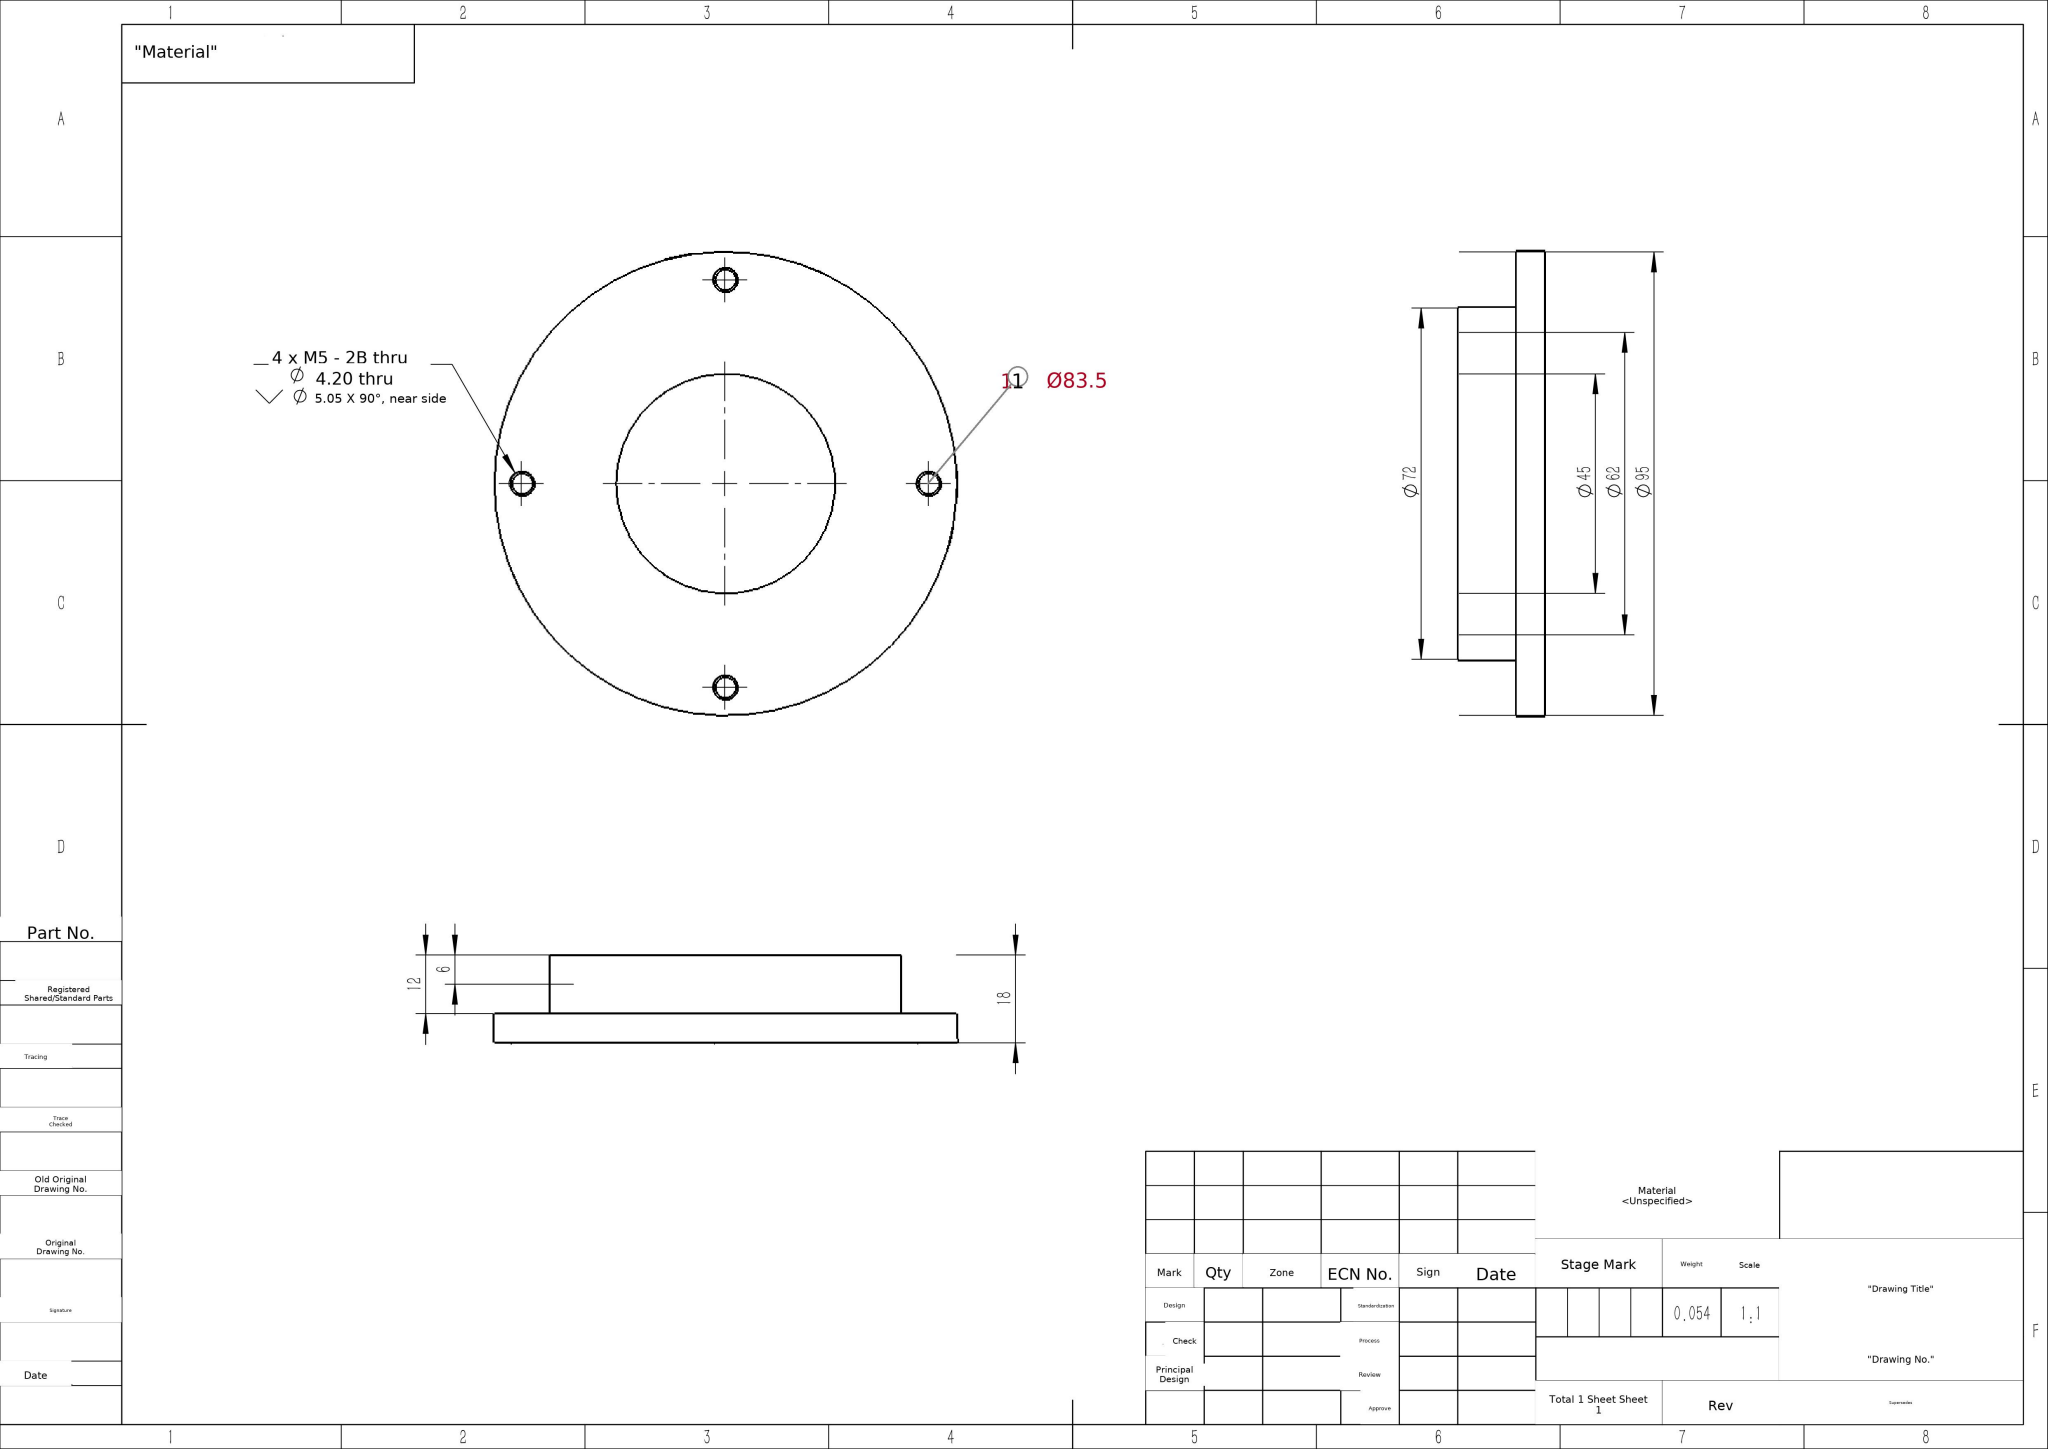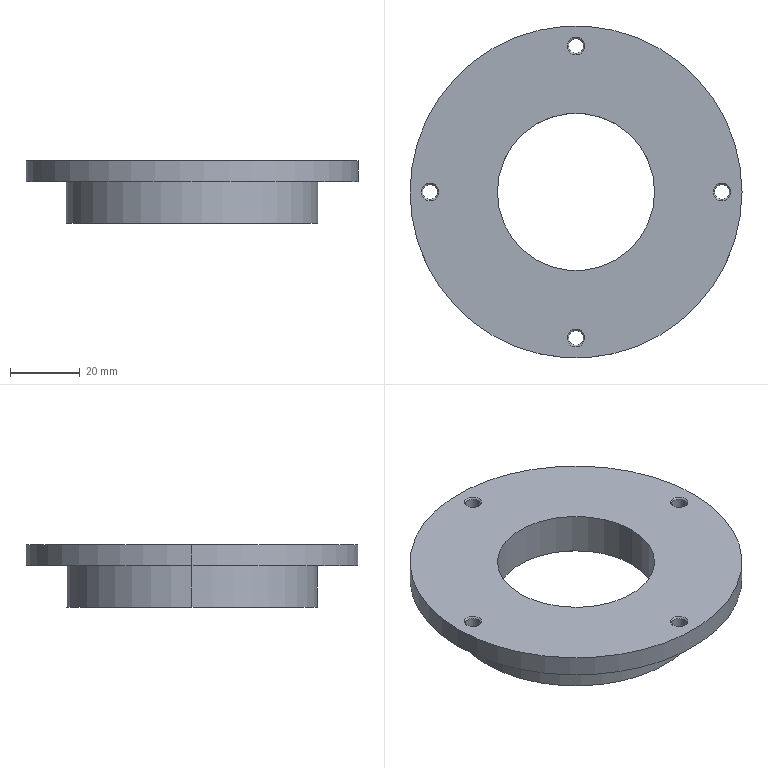Part | SolidWorks | mm | 1 solid | 28 faces | box 95 x 95 x 18 mm | volume 53850 mm3 | cylinder 16 | cone 8 | plane 4 | commonest cylinder face diameters 4.2 x8 62 x2 72 x2 95 x2 45 x2
build123d program:
from build123d import *

# Parameters (mm, degrees)
SKETCH1_R                   = 47.5
BOSS_EXTRUDE1_DEPTH         = 18
SKETCH2_R                   = 47.5
SKETCH2_R_2                 = 36
CUT_EXTRUDE1_DEPTH          = 12
SKETCH3_R                   = 22.5
CUT_EXTRUDE2_DEPTH          = 30
M5_TAPPED_HOLE1_D           = 4.2
M5_TAPPED_HOLE1_CSINK_D     = 5.05
M5_TAPPED_HOLE1_CSINK_ANGLE = 90
SKETCH6_R                   = 31
SKETCH6_R_2                 = 22.5
CUT_EXTRUDE3_DEPTH          = 6


with BuildPart() as part:
    # Sketch1 → Boss-Extrude1 (new body)
    with BuildSketch(Plane.XY):
        Circle(SKETCH1_R)
    extrude(amount=BOSS_EXTRUDE1_DEPTH)

    # Sketch2 → Cut-Extrude1 (cut)
    with BuildSketch(Plane(origin=(0, 0, 0), x_dir=(-1, 0, 0), z_dir=(0, 0, -1))):
        Circle(SKETCH2_R)
        Circle(SKETCH2_R_2, mode=Mode.SUBTRACT)
    extrude(amount=-CUT_EXTRUDE1_DEPTH, mode=Mode.SUBTRACT)

    # Sketch3 → Cut-Extrude2 (cut)
    with BuildSketch(Plane(origin=(0, 0, 0), x_dir=(-1, 0, 0), z_dir=(0, 0, -1))):
        Circle(SKETCH3_R)
    extrude(amount=-CUT_EXTRUDE2_DEPTH, mode=Mode.SUBTRACT)

    # M5 Tapped Hole1 (through all)
    with Locations(Plane(origin=(-41.75, 0, 18), x_dir=(1, 0, 0), z_dir=(0, 0, 1))):
        with Locations((0, 0), (41.75, 41.75), (83.5, 0), (41.75, -41.75)):
            CounterSinkHole(M5_TAPPED_HOLE1_D / 2, M5_TAPPED_HOLE1_CSINK_D / 2, counter_sink_angle=M5_TAPPED_HOLE1_CSINK_ANGLE)

    # Sketch6 → Cut-Extrude3 (cut)
    with BuildSketch(Plane(origin=(0, 0, 0), x_dir=(-1, 0, 0), z_dir=(0, 0, -1))):
        Circle(SKETCH6_R)
        Circle(SKETCH6_R_2, mode=Mode.SUBTRACT)
    extrude(amount=-CUT_EXTRUDE3_DEPTH, mode=Mode.SUBTRACT)


solid = part.part
STEP:
#1=CARTESIAN_POINT('',(31.,0.,6.));
#2=VERTEX_POINT('',#1);
#3=CARTESIAN_POINT('',(-31.,0.,6.));
#4=VERTEX_POINT('',#3);
#5=CARTESIAN_POINT('',(0.,0.,6.));
#6=DIRECTION('',(0.,0.,-1.));
#7=DIRECTION('',(-1.,0.,0.));
#8=AXIS2_PLACEMENT_3D('',#5,#6,#7);
#9=CIRCLE('',#8,31.);
#10=EDGE_CURVE('',#2,#4,#9,.T.);
#11=ORIENTED_EDGE('',*,*,#10,.F.);
#12=CARTESIAN_POINT('',(31.,0.,0.));
#13=VERTEX_POINT('',#12);
#14=CARTESIAN_POINT('',(31.,0.,6.));
#15=DIRECTION('',(0.,0.,-1.));
#16=VECTOR('',#15,1000.);
#17=LINE('',#14,#16);
#18=EDGE_CURVE('',#2,#13,#17,.T.);
#19=ORIENTED_EDGE('',*,*,#18,.T.);
#20=CARTESIAN_POINT('',(-31.,0.,0.));
#21=VERTEX_POINT('',#20);
#22=CARTESIAN_POINT('',(0.,0.,0.));
#23=DIRECTION('',(0.,0.,-1.));
#24=DIRECTION('',(-1.,0.,0.));
#25=AXIS2_PLACEMENT_3D('',#22,#23,#24);
#26=CIRCLE('',#25,31.);
#27=EDGE_CURVE('',#13,#21,#26,.T.);
#28=ORIENTED_EDGE('',*,*,#27,.T.);
#29=CARTESIAN_POINT('',(-31.,0.,6.));
#30=DIRECTION('',(0.,0.,-1.));
#31=VECTOR('',#30,1000.);
#32=LINE('',#29,#31);
#33=EDGE_CURVE('',#4,#21,#32,.T.);
#34=ORIENTED_EDGE('',*,*,#33,.F.);
#35=EDGE_LOOP('',(#11,#19,#28,#34));
#36=FACE_OUTER_BOUND('',#35,.T.);
#37=CARTESIAN_POINT('',(0.,0.,6.));
#38=DIRECTION('',(0.,0.,-1.));
#39=DIRECTION('',(-1.,0.,0.));
#40=AXIS2_PLACEMENT_3D('',#37,#38,#39);
#41=CYLINDRICAL_SURFACE('',#40,31.);
#42=ADVANCED_FACE('',(#36),#41,.F.);
#43=CARTESIAN_POINT('',(-43.85,0.,17.575));
#44=VERTEX_POINT('',#43);
#45=CARTESIAN_POINT('',(-39.65,0.,17.575));
#46=VERTEX_POINT('',#45);
#47=CARTESIAN_POINT('',(-41.75,0.,17.575));
#48=DIRECTION('',(0.,0.,1.));
#49=DIRECTION('',(1.,0.,0.));
#50=AXIS2_PLACEMENT_3D('',#47,#48,#49);
#51=CIRCLE('',#50,2.1);
#52=EDGE_CURVE('',#44,#46,#51,.T.);
#53=ORIENTED_EDGE('',*,*,#52,.F.);
#54=CARTESIAN_POINT('',(-44.275,0.,18.));
#55=VERTEX_POINT('',#54);
#56=CARTESIAN_POINT('',(-44.275,0.,18.));
#57=DIRECTION('',(-0.7071,0.,0.7071));
#58=VECTOR('',#57,1000.);
#59=LINE('',#56,#58);
#60=EDGE_CURVE('',#44,#55,#59,.T.);
#61=ORIENTED_EDGE('',*,*,#60,.T.);
#62=CARTESIAN_POINT('',(-39.225,0.,18.));
#63=VERTEX_POINT('',#62);
#64=CARTESIAN_POINT('',(-41.75,0.,18.));
#65=DIRECTION('',(0.,0.,1.));
#66=DIRECTION('',(1.,0.,0.));
#67=AXIS2_PLACEMENT_3D('',#64,#65,#66);
#68=CIRCLE('',#67,2.525);
#69=EDGE_CURVE('',#55,#63,#68,.T.);
#70=ORIENTED_EDGE('',*,*,#69,.T.);
#71=CARTESIAN_POINT('',(-39.225,0.,18.));
#72=DIRECTION('',(0.7071,0.,0.7071));
#73=VECTOR('',#72,1000.);
#74=LINE('',#71,#73);
#75=EDGE_CURVE('',#46,#63,#74,.T.);
#76=ORIENTED_EDGE('',*,*,#75,.F.);
#77=EDGE_LOOP('',(#53,#61,#70,#76));
#78=FACE_OUTER_BOUND('',#77,.T.);
#79=CARTESIAN_POINT('',(-41.75,0.,18.));
#80=DIRECTION('',(0.,0.,1.));
#81=DIRECTION('',(1.,0.,0.));
#82=AXIS2_PLACEMENT_3D('',#79,#80,#81);
#83=CONICAL_SURFACE('',#82,2.525,0.7854);
#84=ADVANCED_FACE('',(#78),#83,.F.);
#85=CARTESIAN_POINT('',(-39.65,0.,12.));
#86=VERTEX_POINT('',#85);
#87=CARTESIAN_POINT('',(-43.85,0.,12.));
#88=VERTEX_POINT('',#87);
#89=CARTESIAN_POINT('',(-41.75,0.,12.));
#90=DIRECTION('',(0.,0.,-1.));
#91=DIRECTION('',(-1.,0.,0.));
#92=AXIS2_PLACEMENT_3D('',#89,#90,#91);
#93=CIRCLE('',#92,2.1);
#94=EDGE_CURVE('',#86,#88,#93,.T.);
#95=ORIENTED_EDGE('',*,*,#94,.T.);
#96=CARTESIAN_POINT('',(-43.85,0.,18.));
#97=DIRECTION('',(0.,0.,1.));
#98=VECTOR('',#97,1000.);
#99=LINE('',#96,#98);
#100=EDGE_CURVE('',#88,#44,#99,.T.);
#101=ORIENTED_EDGE('',*,*,#100,.T.);
#102=ORIENTED_EDGE('',*,*,#52,.T.);
#103=CARTESIAN_POINT('',(-39.65,0.,18.));
#104=DIRECTION('',(0.,0.,1.));
#105=VECTOR('',#104,1000.);
#106=LINE('',#103,#105);
#107=EDGE_CURVE('',#86,#46,#106,.T.);
#108=ORIENTED_EDGE('',*,*,#107,.F.);
#109=EDGE_LOOP('',(#95,#101,#102,#108));
#110=FACE_OUTER_BOUND('',#109,.T.);
#111=CARTESIAN_POINT('',(-41.75,0.,18.));
#112=DIRECTION('',(0.,0.,1.));
#113=DIRECTION('',(1.,0.,0.));
#114=AXIS2_PLACEMENT_3D('',#111,#112,#113);
#115=CYLINDRICAL_SURFACE('',#114,2.1);
#116=ADVANCED_FACE('',(#110),#115,.F.);
#117=CARTESIAN_POINT('',(-2.1,41.75,17.575));
#118=VERTEX_POINT('',#117);
#119=CARTESIAN_POINT('',(2.1,41.75,17.575));
#120=VERTEX_POINT('',#119);
#121=CARTESIAN_POINT('',(0.,41.75,17.575));
#122=DIRECTION('',(0.,0.,1.));
#123=DIRECTION('',(1.,0.,0.));
#124=AXIS2_PLACEMENT_3D('',#121,#122,#123);
#125=CIRCLE('',#124,2.1);
#126=EDGE_CURVE('',#118,#120,#125,.T.);
#127=ORIENTED_EDGE('',*,*,#126,.F.);
#128=CARTESIAN_POINT('',(-2.525,41.75,18.));
#129=VERTEX_POINT('',#128);
#130=CARTESIAN_POINT('',(-2.525,41.75,18.));
#131=DIRECTION('',(-0.7071,0.,0.7071));
#132=VECTOR('',#131,1000.);
#133=LINE('',#130,#132);
#134=EDGE_CURVE('',#118,#129,#133,.T.);
#135=ORIENTED_EDGE('',*,*,#134,.T.);
#136=CARTESIAN_POINT('',(2.525,41.75,18.));
#137=VERTEX_POINT('',#136);
#138=CARTESIAN_POINT('',(0.,41.75,18.));
#139=DIRECTION('',(0.,0.,1.));
#140=DIRECTION('',(1.,0.,0.));
#141=AXIS2_PLACEMENT_3D('',#138,#139,#140);
#142=CIRCLE('',#141,2.525);
#143=EDGE_CURVE('',#129,#137,#142,.T.);
#144=ORIENTED_EDGE('',*,*,#143,.T.);
#145=CARTESIAN_POINT('',(2.525,41.75,18.));
#146=DIRECTION('',(0.7071,0.,0.7071));
#147=VECTOR('',#146,1000.);
#148=LINE('',#145,#147);
#149=EDGE_CURVE('',#120,#137,#148,.T.);
#150=ORIENTED_EDGE('',*,*,#149,.F.);
#151=EDGE_LOOP('',(#127,#135,#144,#150));
#152=FACE_OUTER_BOUND('',#151,.T.);
#153=CARTESIAN_POINT('',(0.,41.75,18.));
#154=DIRECTION('',(0.,0.,1.));
#155=DIRECTION('',(1.,0.,0.));
#156=AXIS2_PLACEMENT_3D('',#153,#154,#155);
#157=CONICAL_SURFACE('',#156,2.525,0.7854);
#158=ADVANCED_FACE('',(#152),#157,.F.);
#159=CARTESIAN_POINT('',(2.1,41.75,12.));
#160=VERTEX_POINT('',#159);
#161=CARTESIAN_POINT('',(-2.1,41.75,12.));
#162=VERTEX_POINT('',#161);
#163=CARTESIAN_POINT('',(0.,41.75,12.));
#164=DIRECTION('',(0.,0.,-1.));
#165=DIRECTION('',(-1.,0.,0.));
#166=AXIS2_PLACEMENT_3D('',#163,#164,#165);
#167=CIRCLE('',#166,2.1);
#168=EDGE_CURVE('',#160,#162,#167,.T.);
#169=ORIENTED_EDGE('',*,*,#168,.T.);
#170=CARTESIAN_POINT('',(-2.1,41.75,18.));
#171=DIRECTION('',(0.,0.,1.));
#172=VECTOR('',#171,1000.);
#173=LINE('',#170,#172);
#174=EDGE_CURVE('',#162,#118,#173,.T.);
#175=ORIENTED_EDGE('',*,*,#174,.T.);
#176=ORIENTED_EDGE('',*,*,#126,.T.);
#177=CARTESIAN_POINT('',(2.1,41.75,18.));
#178=DIRECTION('',(0.,0.,1.));
#179=VECTOR('',#178,1000.);
#180=LINE('',#177,#179);
#181=EDGE_CURVE('',#160,#120,#180,.T.);
#182=ORIENTED_EDGE('',*,*,#181,.F.);
#183=EDGE_LOOP('',(#169,#175,#176,#182));
#184=FACE_OUTER_BOUND('',#183,.T.);
#185=CARTESIAN_POINT('',(0.,41.75,18.));
#186=DIRECTION('',(0.,0.,1.));
#187=DIRECTION('',(1.,0.,0.));
#188=AXIS2_PLACEMENT_3D('',#185,#186,#187);
#189=CYLINDRICAL_SURFACE('',#188,2.1);
#190=ADVANCED_FACE('',(#184),#189,.F.);
#191=CARTESIAN_POINT('',(39.65,0.,17.575));
#192=VERTEX_POINT('',#191);
#193=CARTESIAN_POINT('',(43.85,0.,17.575));
#194=VERTEX_POINT('',#193);
#195=CARTESIAN_POINT('',(41.75,0.,17.575));
#196=DIRECTION('',(0.,0.,1.));
#197=DIRECTION('',(1.,0.,0.));
#198=AXIS2_PLACEMENT_3D('',#195,#196,#197);
#199=CIRCLE('',#198,2.1);
#200=EDGE_CURVE('',#192,#194,#199,.T.);
#201=ORIENTED_EDGE('',*,*,#200,.F.);
#202=CARTESIAN_POINT('',(39.225,0.,18.));
#203=VERTEX_POINT('',#202);
#204=CARTESIAN_POINT('',(39.225,0.,18.));
#205=DIRECTION('',(-0.7071,0.,0.7071));
#206=VECTOR('',#205,1000.);
#207=LINE('',#204,#206);
#208=EDGE_CURVE('',#192,#203,#207,.T.);
#209=ORIENTED_EDGE('',*,*,#208,.T.);
#210=CARTESIAN_POINT('',(44.275,0.,18.));
#211=VERTEX_POINT('',#210);
#212=CARTESIAN_POINT('',(41.75,0.,18.));
#213=DIRECTION('',(0.,0.,1.));
#214=DIRECTION('',(1.,0.,0.));
#215=AXIS2_PLACEMENT_3D('',#212,#213,#214);
#216=CIRCLE('',#215,2.525);
#217=EDGE_CURVE('',#203,#211,#216,.T.);
#218=ORIENTED_EDGE('',*,*,#217,.T.);
#219=CARTESIAN_POINT('',(44.275,0.,18.));
#220=DIRECTION('',(0.7071,0.,0.7071));
#221=VECTOR('',#220,1000.);
#222=LINE('',#219,#221);
#223=EDGE_CURVE('',#194,#211,#222,.T.);
#224=ORIENTED_EDGE('',*,*,#223,.F.);
#225=EDGE_LOOP('',(#201,#209,#218,#224));
#226=FACE_OUTER_BOUND('',#225,.T.);
#227=CARTESIAN_POINT('',(41.75,0.,18.));
#228=DIRECTION('',(0.,0.,1.));
#229=DIRECTION('',(1.,0.,0.));
#230=AXIS2_PLACEMENT_3D('',#227,#228,#229);
#231=CONICAL_SURFACE('',#230,2.525,0.7854);
#232=ADVANCED_FACE('',(#226),#231,.F.);
#233=CARTESIAN_POINT('',(43.85,0.,12.));
#234=VERTEX_POINT('',#233);
#235=CARTESIAN_POINT('',(39.65,0.,12.));
#236=VERTEX_POINT('',#235);
#237=CARTESIAN_POINT('',(41.75,0.,12.));
#238=DIRECTION('',(0.,0.,-1.));
#239=DIRECTION('',(-1.,0.,0.));
#240=AXIS2_PLACEMENT_3D('',#237,#238,#239);
#241=CIRCLE('',#240,2.1);
#242=EDGE_CURVE('',#234,#236,#241,.T.);
#243=ORIENTED_EDGE('',*,*,#242,.T.);
#244=CARTESIAN_POINT('',(39.65,0.,18.));
#245=DIRECTION('',(0.,0.,1.));
#246=VECTOR('',#245,1000.);
#247=LINE('',#244,#246);
#248=EDGE_CURVE('',#236,#192,#247,.T.);
#249=ORIENTED_EDGE('',*,*,#248,.T.);
#250=ORIENTED_EDGE('',*,*,#200,.T.);
#251=CARTESIAN_POINT('',(43.85,0.,18.));
#252=DIRECTION('',(0.,0.,1.));
#253=VECTOR('',#252,1000.);
#254=LINE('',#251,#253);
#255=EDGE_CURVE('',#234,#194,#254,.T.);
#256=ORIENTED_EDGE('',*,*,#255,.F.);
#257=EDGE_LOOP('',(#243,#249,#250,#256));
#258=FACE_OUTER_BOUND('',#257,.T.);
#259=CARTESIAN_POINT('',(41.75,0.,18.));
#260=DIRECTION('',(0.,0.,1.));
#261=DIRECTION('',(1.,0.,0.));
#262=AXIS2_PLACEMENT_3D('',#259,#260,#261);
#263=CYLINDRICAL_SURFACE('',#262,2.1);
#264=ADVANCED_FACE('',(#258),#263,.F.);
#265=CARTESIAN_POINT('',(-2.1,-41.75,17.575));
#266=VERTEX_POINT('',#265);
#267=CARTESIAN_POINT('',(2.1,-41.75,17.575));
#268=VERTEX_POINT('',#267);
#269=CARTESIAN_POINT('',(0.,-41.75,17.575));
#270=DIRECTION('',(0.,0.,1.));
#271=DIRECTION('',(1.,0.,0.));
#272=AXIS2_PLACEMENT_3D('',#269,#270,#271);
#273=CIRCLE('',#272,2.1);
#274=EDGE_CURVE('',#266,#268,#273,.T.);
#275=ORIENTED_EDGE('',*,*,#274,.F.);
#276=CARTESIAN_POINT('',(-2.525,-41.75,18.));
#277=VERTEX_POINT('',#276);
#278=CARTESIAN_POINT('',(-2.525,-41.75,18.));
#279=DIRECTION('',(-0.7071,0.,0.7071));
#280=VECTOR('',#279,1000.);
#281=LINE('',#278,#280);
#282=EDGE_CURVE('',#266,#277,#281,.T.);
#283=ORIENTED_EDGE('',*,*,#282,.T.);
#284=CARTESIAN_POINT('',(2.525,-41.75,18.));
#285=VERTEX_POINT('',#284);
#286=CARTESIAN_POINT('',(0.,-41.75,18.));
#287=DIRECTION('',(0.,0.,1.));
#288=DIRECTION('',(1.,0.,0.));
#289=AXIS2_PLACEMENT_3D('',#286,#287,#288);
#290=CIRCLE('',#289,2.525);
#291=EDGE_CURVE('',#277,#285,#290,.T.);
#292=ORIENTED_EDGE('',*,*,#291,.T.);
#293=CARTESIAN_POINT('',(2.525,-41.75,18.));
#294=DIRECTION('',(0.7071,0.,0.7071));
#295=VECTOR('',#294,1000.);
#296=LINE('',#293,#295);
#297=EDGE_CURVE('',#268,#285,#296,.T.);
#298=ORIENTED_EDGE('',*,*,#297,.F.);
#299=EDGE_LOOP('',(#275,#283,#292,#298));
#300=FACE_OUTER_BOUND('',#299,.T.);
#301=CARTESIAN_POINT('',(0.,-41.75,18.));
#302=DIRECTION('',(0.,0.,1.));
#303=DIRECTION('',(1.,0.,0.));
#304=AXIS2_PLACEMENT_3D('',#301,#302,#303);
#305=CONICAL_SURFACE('',#304,2.525,0.7854);
#306=ADVANCED_FACE('',(#300),#305,.F.);
#307=CARTESIAN_POINT('',(2.1,-41.75,12.));
#308=VERTEX_POINT('',#307);
#309=CARTESIAN_POINT('',(-2.1,-41.75,12.));
#310=VERTEX_POINT('',#309);
#311=CARTESIAN_POINT('',(0.,-41.75,12.));
#312=DIRECTION('',(0.,0.,-1.));
#313=DIRECTION('',(-1.,0.,0.));
#314=AXIS2_PLACEMENT_3D('',#311,#312,#313);
#315=CIRCLE('',#314,2.1);
#316=EDGE_CURVE('',#308,#310,#315,.T.);
#317=ORIENTED_EDGE('',*,*,#316,.T.);
#318=CARTESIAN_POINT('',(-2.1,-41.75,18.));
#319=DIRECTION('',(0.,0.,1.));
#320=VECTOR('',#319,1000.);
#321=LINE('',#318,#320);
#322=EDGE_CURVE('',#310,#266,#321,.T.);
#323=ORIENTED_EDGE('',*,*,#322,.T.);
#324=ORIENTED_EDGE('',*,*,#274,.T.);
#325=CARTESIAN_POINT('',(2.1,-41.75,18.));
#326=DIRECTION('',(0.,0.,1.));
#327=VECTOR('',#326,1000.);
#328=LINE('',#325,#327);
#329=EDGE_CURVE('',#308,#268,#328,.T.);
#330=ORIENTED_EDGE('',*,*,#329,.F.);
#331=EDGE_LOOP('',(#317,#323,#324,#330));
#332=FACE_OUTER_BOUND('',#331,.T.);
#333=CARTESIAN_POINT('',(0.,-41.75,18.));
#334=DIRECTION('',(0.,0.,1.));
#335=DIRECTION('',(1.,0.,0.));
#336=AXIS2_PLACEMENT_3D('',#333,#334,#335);
#337=CYLINDRICAL_SURFACE('',#336,2.1);
#338=ADVANCED_FACE('',(#332),#337,.F.);
#339=CARTESIAN_POINT('',(-36.,0.,12.));
#340=VERTEX_POINT('',#339);
#341=CARTESIAN_POINT('',(36.,0.,12.));
#342=VERTEX_POINT('',#341);
#343=CARTESIAN_POINT('',(0.,0.,12.));
#344=DIRECTION('',(0.,0.,-1.));
#345=DIRECTION('',(-1.,0.,0.));
#346=AXIS2_PLACEMENT_3D('',#343,#344,#345);
#347=CIRCLE('',#346,36.);
#348=EDGE_CURVE('',#340,#342,#347,.T.);
#349=ORIENTED_EDGE('',*,*,#348,.T.);
#350=CARTESIAN_POINT('',(36.,0.,0.));
#351=VERTEX_POINT('',#350);
#352=CARTESIAN_POINT('',(36.,0.,12.));
#353=DIRECTION('',(0.,0.,-1.));
#354=VECTOR('',#353,1000.);
#355=LINE('',#352,#354);
#356=EDGE_CURVE('',#342,#351,#355,.T.);
#357=ORIENTED_EDGE('',*,*,#356,.T.);
#358=CARTESIAN_POINT('',(-36.,0.,0.));
#359=VERTEX_POINT('',#358);
#360=CARTESIAN_POINT('',(0.,0.,0.));
#361=DIRECTION('',(0.,0.,-1.));
#362=DIRECTION('',(-1.,0.,0.));
#363=AXIS2_PLACEMENT_3D('',#360,#361,#362);
#364=CIRCLE('',#363,36.);
#365=EDGE_CURVE('',#359,#351,#364,.T.);
#366=ORIENTED_EDGE('',*,*,#365,.F.);
#367=CARTESIAN_POINT('',(-36.,0.,12.));
#368=DIRECTION('',(0.,0.,-1.));
#369=VECTOR('',#368,1000.);
#370=LINE('',#367,#369);
#371=EDGE_CURVE('',#340,#359,#370,.T.);
#372=ORIENTED_EDGE('',*,*,#371,.F.);
#373=EDGE_LOOP('',(#349,#357,#366,#372));
#374=FACE_OUTER_BOUND('',#373,.T.);
#375=CARTESIAN_POINT('',(0.,0.,12.));
#376=DIRECTION('',(0.,0.,-1.));
#377=DIRECTION('',(-1.,0.,0.));
#378=AXIS2_PLACEMENT_3D('',#375,#376,#377);
#379=CYLINDRICAL_SURFACE('',#378,36.);
#380=ADVANCED_FACE('',(#374),#379,.T.);
#381=CARTESIAN_POINT('',(47.5,0.,18.));
#382=VERTEX_POINT('',#381);
#383=CARTESIAN_POINT('',(-47.5,0.,18.));
#384=VERTEX_POINT('',#383);
#385=CARTESIAN_POINT('',(0.,0.,18.));
#386=DIRECTION('',(0.,0.,1.));
#387=DIRECTION('',(1.,0.,0.));
#388=AXIS2_PLACEMENT_3D('',#385,#386,#387);
#389=CIRCLE('',#388,47.5);
#390=EDGE_CURVE('',#382,#384,#389,.T.);
#391=ORIENTED_EDGE('',*,*,#390,.F.);
#392=CARTESIAN_POINT('',(47.5,0.,12.));
#393=VERTEX_POINT('',#392);
#394=CARTESIAN_POINT('',(47.5,0.,18.));
#395=DIRECTION('',(0.,0.,-1.));
#396=VECTOR('',#395,1000.);
#397=LINE('',#394,#396);
#398=EDGE_CURVE('',#382,#393,#397,.T.);
#399=ORIENTED_EDGE('',*,*,#398,.T.);
#400=CARTESIAN_POINT('',(-47.5,0.,12.));
#401=VERTEX_POINT('',#400);
#402=CARTESIAN_POINT('',(0.,0.,12.));
#403=DIRECTION('',(0.,0.,-1.));
#404=DIRECTION('',(-1.,0.,0.));
#405=AXIS2_PLACEMENT_3D('',#402,#403,#404);
#406=CIRCLE('',#405,47.5);
#407=EDGE_CURVE('',#401,#393,#406,.T.);
#408=ORIENTED_EDGE('',*,*,#407,.F.);
#409=CARTESIAN_POINT('',(-47.5,0.,18.));
#410=DIRECTION('',(0.,0.,-1.));
#411=VECTOR('',#410,1000.);
#412=LINE('',#409,#411);
#413=EDGE_CURVE('',#384,#401,#412,.T.);
#414=ORIENTED_EDGE('',*,*,#413,.F.);
#415=EDGE_LOOP('',(#391,#399,#408,#414));
#416=FACE_OUTER_BOUND('',#415,.T.);
#417=CARTESIAN_POINT('',(0.,0.,18.));
#418=DIRECTION('',(0.,0.,-1.));
#419=DIRECTION('',(-1.,0.,0.));
#420=AXIS2_PLACEMENT_3D('',#417,#418,#419);
#421=CYLINDRICAL_SURFACE('',#420,47.5);
#422=ADVANCED_FACE('',(#416),#421,.T.);
#423=CARTESIAN_POINT('',(-22.5,0.,18.));
#424=VERTEX_POINT('',#423);
#425=CARTESIAN_POINT('',(22.5,0.,18.));
#426=VERTEX_POINT('',#425);
#427=CARTESIAN_POINT('',(0.,0.,18.));
#428=DIRECTION('',(0.,0.,1.));
#429=DIRECTION('',(1.,0.,0.));
#430=AXIS2_PLACEMENT_3D('',#427,#428,#429);
#431=CIRCLE('',#430,22.5);
#432=EDGE_CURVE('',#424,#426,#431,.T.);
#433=ORIENTED_EDGE('',*,*,#432,.T.);
#434=CARTESIAN_POINT('',(22.5,0.,6.));
#435=VERTEX_POINT('',#434);
#436=CARTESIAN_POINT('',(22.5,0.,30.));
#437=DIRECTION('',(0.,0.,-1.));
#438=VECTOR('',#437,1000.);
#439=LINE('',#436,#438);
#440=EDGE_CURVE('',#426,#435,#439,.T.);
#441=ORIENTED_EDGE('',*,*,#440,.T.);
#442=CARTESIAN_POINT('',(-22.5,0.,6.));
#443=VERTEX_POINT('',#442);
#444=CARTESIAN_POINT('',(0.,0.,6.));
#445=DIRECTION('',(0.,0.,-1.));
#446=DIRECTION('',(-1.,0.,0.));
#447=AXIS2_PLACEMENT_3D('',#444,#445,#446);
#448=CIRCLE('',#447,22.5);
#449=EDGE_CURVE('',#435,#443,#448,.T.);
#450=ORIENTED_EDGE('',*,*,#449,.T.);
#451=CARTESIAN_POINT('',(-22.5,0.,30.));
#452=DIRECTION('',(0.,0.,-1.));
#453=VECTOR('',#452,1000.);
#454=LINE('',#451,#453);
#455=EDGE_CURVE('',#424,#443,#454,.T.);
#456=ORIENTED_EDGE('',*,*,#455,.F.);
#457=EDGE_LOOP('',(#433,#441,#450,#456));
#458=FACE_OUTER_BOUND('',#457,.T.);
#459=CARTESIAN_POINT('',(0.,0.,30.));
#460=DIRECTION('',(0.,0.,-1.));
#461=DIRECTION('',(-1.,0.,0.));
#462=AXIS2_PLACEMENT_3D('',#459,#460,#461);
#463=CYLINDRICAL_SURFACE('',#462,22.5);
#464=ADVANCED_FACE('',(#458),#463,.F.);
#465=ORIENTED_EDGE('',*,*,#440,.F.);
#466=CARTESIAN_POINT('',(0.,0.,18.));
#467=DIRECTION('',(0.,0.,1.));
#468=DIRECTION('',(1.,0.,0.));
#469=AXIS2_PLACEMENT_3D('',#466,#467,#468);
#470=CIRCLE('',#469,22.5);
#471=EDGE_CURVE('',#426,#424,#470,.T.);
#472=ORIENTED_EDGE('',*,*,#471,.T.);
#473=ORIENTED_EDGE('',*,*,#455,.T.);
#474=CARTESIAN_POINT('',(0.,0.,6.));
#475=DIRECTION('',(0.,0.,-1.));
#476=DIRECTION('',(-1.,0.,0.));
#477=AXIS2_PLACEMENT_3D('',#474,#475,#476);
#478=CIRCLE('',#477,22.5);
#479=EDGE_CURVE('',#443,#435,#478,.T.);
#480=ORIENTED_EDGE('',*,*,#479,.T.);
#481=EDGE_LOOP('',(#465,#472,#473,#480));
#482=FACE_OUTER_BOUND('',#481,.T.);
#483=CARTESIAN_POINT('',(0.,0.,30.));
#484=DIRECTION('',(0.,0.,-1.));
#485=DIRECTION('',(-1.,0.,0.));
#486=AXIS2_PLACEMENT_3D('',#483,#484,#485);
#487=CYLINDRICAL_SURFACE('',#486,22.5);
#488=ADVANCED_FACE('',(#482),#487,.F.);
#489=ORIENTED_EDGE('',*,*,#398,.F.);
#490=CARTESIAN_POINT('',(0.,0.,18.));
#491=DIRECTION('',(0.,0.,1.));
#492=DIRECTION('',(1.,0.,0.));
#493=AXIS2_PLACEMENT_3D('',#490,#491,#492);
#494=CIRCLE('',#493,47.5);
#495=EDGE_CURVE('',#384,#382,#494,.T.);
#496=ORIENTED_EDGE('',*,*,#495,.F.);
#497=ORIENTED_EDGE('',*,*,#413,.T.);
#498=CARTESIAN_POINT('',(0.,0.,12.));
#499=DIRECTION('',(0.,0.,-1.));
#500=DIRECTION('',(-1.,0.,0.));
#501=AXIS2_PLACEMENT_3D('',#498,#499,#500);
#502=CIRCLE('',#501,47.5);
#503=EDGE_CURVE('',#393,#401,#502,.T.);
#504=ORIENTED_EDGE('',*,*,#503,.F.);
#505=EDGE_LOOP('',(#489,#496,#497,#504));
#506=FACE_OUTER_BOUND('',#505,.T.);
#507=CARTESIAN_POINT('',(0.,0.,18.));
#508=DIRECTION('',(0.,0.,-1.));
#509=DIRECTION('',(-1.,0.,0.));
#510=AXIS2_PLACEMENT_3D('',#507,#508,#509);
#511=CYLINDRICAL_SURFACE('',#510,47.5);
#512=ADVANCED_FACE('',(#506),#511,.T.);
#513=CARTESIAN_POINT('',(-41.75,0.,18.));
#514=DIRECTION('',(0.,0.,1.));
#515=DIRECTION('',(1.,0.,0.));
#516=AXIS2_PLACEMENT_3D('',#513,#514,#515);
#517=CIRCLE('',#516,2.525);
#518=EDGE_CURVE('',#63,#55,#517,.T.);
#519=ORIENTED_EDGE('',*,*,#518,.F.);
#520=ORIENTED_EDGE('',*,*,#69,.F.);
#521=EDGE_LOOP('',(#519,#520));
#522=FACE_BOUND('',#521,.T.);
#523=CARTESIAN_POINT('',(0.,41.75,18.));
#524=DIRECTION('',(0.,0.,1.));
#525=DIRECTION('',(1.,0.,0.));
#526=AXIS2_PLACEMENT_3D('',#523,#524,#525);
#527=CIRCLE('',#526,2.525);
#528=EDGE_CURVE('',#137,#129,#527,.T.);
#529=ORIENTED_EDGE('',*,*,#528,.F.);
#530=ORIENTED_EDGE('',*,*,#143,.F.);
#531=EDGE_LOOP('',(#529,#530));
#532=FACE_BOUND('',#531,.T.);
#533=CARTESIAN_POINT('',(41.75,0.,18.));
#534=DIRECTION('',(0.,0.,1.));
#535=DIRECTION('',(1.,0.,0.));
#536=AXIS2_PLACEMENT_3D('',#533,#534,#535);
#537=CIRCLE('',#536,2.525);
#538=EDGE_CURVE('',#211,#203,#537,.T.);
#539=ORIENTED_EDGE('',*,*,#538,.F.);
#540=ORIENTED_EDGE('',*,*,#217,.F.);
#541=EDGE_LOOP('',(#539,#540));
#542=FACE_BOUND('',#541,.T.);
#543=CARTESIAN_POINT('',(0.,-41.75,18.));
#544=DIRECTION('',(0.,0.,1.));
#545=DIRECTION('',(1.,0.,0.));
#546=AXIS2_PLACEMENT_3D('',#543,#544,#545);
#547=CIRCLE('',#546,2.525);
#548=EDGE_CURVE('',#285,#277,#547,.T.);
#549=ORIENTED_EDGE('',*,*,#548,.F.);
#550=ORIENTED_EDGE('',*,*,#291,.F.);
#551=EDGE_LOOP('',(#549,#550));
#552=FACE_BOUND('',#551,.T.);
#553=ORIENTED_EDGE('',*,*,#432,.F.);
#554=ORIENTED_EDGE('',*,*,#471,.F.);
#555=EDGE_LOOP('',(#553,#554));
#556=FACE_BOUND('',#555,.T.);
#557=ORIENTED_EDGE('',*,*,#495,.T.);
#558=ORIENTED_EDGE('',*,*,#390,.T.);
#559=EDGE_LOOP('',(#557,#558));
#560=FACE_OUTER_BOUND('',#559,.T.);
#561=CARTESIAN_POINT('',(0.,0.,18.));
#562=DIRECTION('',(0.,0.,1.));
#563=DIRECTION('',(1.,0.,0.));
#564=AXIS2_PLACEMENT_3D('',#561,#562,#563);
#565=PLANE('',#564);
#566=ADVANCED_FACE('',(#522,#532,#542,#552,#556,#560),#565,.T.);
#567=ORIENTED_EDGE('',*,*,#94,.F.);
#568=CARTESIAN_POINT('',(-41.75,0.,12.));
#569=DIRECTION('',(0.,0.,-1.));
#570=DIRECTION('',(-1.,0.,0.));
#571=AXIS2_PLACEMENT_3D('',#568,#569,#570);
#572=CIRCLE('',#571,2.1);
#573=EDGE_CURVE('',#88,#86,#572,.T.);
#574=ORIENTED_EDGE('',*,*,#573,.F.);
#575=EDGE_LOOP('',(#567,#574));
#576=FACE_BOUND('',#575,.T.);
#577=ORIENTED_EDGE('',*,*,#168,.F.);
#578=CARTESIAN_POINT('',(0.,41.75,12.));
#579=DIRECTION('',(0.,0.,-1.));
#580=DIRECTION('',(-1.,0.,0.));
#581=AXIS2_PLACEMENT_3D('',#578,#579,#580);
#582=CIRCLE('',#581,2.1);
#583=EDGE_CURVE('',#162,#160,#582,.T.);
#584=ORIENTED_EDGE('',*,*,#583,.F.);
#585=EDGE_LOOP('',(#577,#584));
#586=FACE_BOUND('',#585,.T.);
#587=ORIENTED_EDGE('',*,*,#242,.F.);
#588=CARTESIAN_POINT('',(41.75,0.,12.));
#589=DIRECTION('',(0.,0.,-1.));
#590=DIRECTION('',(-1.,0.,0.));
#591=AXIS2_PLACEMENT_3D('',#588,#589,#590);
#592=CIRCLE('',#591,2.1);
#593=EDGE_CURVE('',#236,#234,#592,.T.);
#594=ORIENTED_EDGE('',*,*,#593,.F.);
#595=EDGE_LOOP('',(#587,#594));
#596=FACE_BOUND('',#595,.T.);
#597=ORIENTED_EDGE('',*,*,#316,.F.);
#598=CARTESIAN_POINT('',(0.,-41.75,12.));
#599=DIRECTION('',(0.,0.,-1.));
#600=DIRECTION('',(-1.,0.,0.));
#601=AXIS2_PLACEMENT_3D('',#598,#599,#600);
#602=CIRCLE('',#601,2.1);
#603=EDGE_CURVE('',#310,#308,#602,.T.);
#604=ORIENTED_EDGE('',*,*,#603,.F.);
#605=EDGE_LOOP('',(#597,#604));
#606=FACE_BOUND('',#605,.T.);
#607=ORIENTED_EDGE('',*,*,#348,.F.);
#608=CARTESIAN_POINT('',(0.,0.,12.));
#609=DIRECTION('',(0.,0.,-1.));
#610=DIRECTION('',(-1.,0.,0.));
#611=AXIS2_PLACEMENT_3D('',#608,#609,#610);
#612=CIRCLE('',#611,36.);
#613=EDGE_CURVE('',#342,#340,#612,.T.);
#614=ORIENTED_EDGE('',*,*,#613,.F.);
#615=EDGE_LOOP('',(#607,#614));
#616=FACE_BOUND('',#615,.T.);
#617=ORIENTED_EDGE('',*,*,#407,.T.);
#618=ORIENTED_EDGE('',*,*,#503,.T.);
#619=EDGE_LOOP('',(#617,#618));
#620=FACE_OUTER_BOUND('',#619,.T.);
#621=CARTESIAN_POINT('',(0.,0.,12.));
#622=DIRECTION('',(0.,0.,-1.));
#623=DIRECTION('',(-1.,0.,0.));
#624=AXIS2_PLACEMENT_3D('',#621,#622,#623);
#625=PLANE('',#624);
#626=ADVANCED_FACE('',(#576,#586,#596,#606,#616,#620),#625,.T.);
#627=ORIENTED_EDGE('',*,*,#356,.F.);
#628=ORIENTED_EDGE('',*,*,#613,.T.);
#629=ORIENTED_EDGE('',*,*,#371,.T.);
#630=CARTESIAN_POINT('',(0.,0.,0.));
#631=DIRECTION('',(0.,0.,-1.));
#632=DIRECTION('',(-1.,0.,0.));
#633=AXIS2_PLACEMENT_3D('',#630,#631,#632);
#634=CIRCLE('',#633,36.);
#635=EDGE_CURVE('',#351,#359,#634,.T.);
#636=ORIENTED_EDGE('',*,*,#635,.F.);
#637=EDGE_LOOP('',(#627,#628,#629,#636));
#638=FACE_OUTER_BOUND('',#637,.T.);
#639=CARTESIAN_POINT('',(0.,0.,12.));
#640=DIRECTION('',(0.,0.,-1.));
#641=DIRECTION('',(-1.,0.,0.));
#642=AXIS2_PLACEMENT_3D('',#639,#640,#641);
#643=CYLINDRICAL_SURFACE('',#642,36.);
#644=ADVANCED_FACE('',(#638),#643,.T.);
#645=CARTESIAN_POINT('',(0.,0.,0.));
#646=DIRECTION('',(0.,0.,-1.));
#647=DIRECTION('',(-1.,0.,0.));
#648=AXIS2_PLACEMENT_3D('',#645,#646,#647);
#649=CIRCLE('',#648,31.);
#650=EDGE_CURVE('',#21,#13,#649,.T.);
#651=ORIENTED_EDGE('',*,*,#650,.F.);
#652=ORIENTED_EDGE('',*,*,#27,.F.);
#653=EDGE_LOOP('',(#651,#652));
#654=FACE_BOUND('',#653,.T.);
#655=ORIENTED_EDGE('',*,*,#365,.T.);
#656=ORIENTED_EDGE('',*,*,#635,.T.);
#657=EDGE_LOOP('',(#655,#656));
#658=FACE_OUTER_BOUND('',#657,.T.);
#659=CARTESIAN_POINT('',(0.,0.,0.));
#660=DIRECTION('',(0.,0.,1.));
#661=DIRECTION('',(1.,0.,0.));
#662=AXIS2_PLACEMENT_3D('',#659,#660,#661);
#663=PLANE('',#662);
#664=ADVANCED_FACE('',(#654,#658),#663,.F.);
#665=ORIENTED_EDGE('',*,*,#322,.F.);
#666=ORIENTED_EDGE('',*,*,#603,.T.);
#667=ORIENTED_EDGE('',*,*,#329,.T.);
#668=CARTESIAN_POINT('',(0.,-41.75,17.575));
#669=DIRECTION('',(0.,0.,1.));
#670=DIRECTION('',(1.,0.,0.));
#671=AXIS2_PLACEMENT_3D('',#668,#669,#670);
#672=CIRCLE('',#671,2.1);
#673=EDGE_CURVE('',#268,#266,#672,.T.);
#674=ORIENTED_EDGE('',*,*,#673,.T.);
#675=EDGE_LOOP('',(#665,#666,#667,#674));
#676=FACE_OUTER_BOUND('',#675,.T.);
#677=CARTESIAN_POINT('',(0.,-41.75,18.));
#678=DIRECTION('',(0.,0.,1.));
#679=DIRECTION('',(1.,0.,0.));
#680=AXIS2_PLACEMENT_3D('',#677,#678,#679);
#681=CYLINDRICAL_SURFACE('',#680,2.1);
#682=ADVANCED_FACE('',(#676),#681,.F.);
#683=ORIENTED_EDGE('',*,*,#282,.F.);
#684=ORIENTED_EDGE('',*,*,#673,.F.);
#685=ORIENTED_EDGE('',*,*,#297,.T.);
#686=ORIENTED_EDGE('',*,*,#548,.T.);
#687=EDGE_LOOP('',(#683,#684,#685,#686));
#688=FACE_OUTER_BOUND('',#687,.T.);
#689=CARTESIAN_POINT('',(0.,-41.75,18.));
#690=DIRECTION('',(0.,0.,1.));
#691=DIRECTION('',(1.,0.,0.));
#692=AXIS2_PLACEMENT_3D('',#689,#690,#691);
#693=CONICAL_SURFACE('',#692,2.525,0.7854);
#694=ADVANCED_FACE('',(#688),#693,.F.);
#695=ORIENTED_EDGE('',*,*,#248,.F.);
#696=ORIENTED_EDGE('',*,*,#593,.T.);
#697=ORIENTED_EDGE('',*,*,#255,.T.);
#698=CARTESIAN_POINT('',(41.75,0.,17.575));
#699=DIRECTION('',(0.,0.,1.));
#700=DIRECTION('',(1.,0.,0.));
#701=AXIS2_PLACEMENT_3D('',#698,#699,#700);
#702=CIRCLE('',#701,2.1);
#703=EDGE_CURVE('',#194,#192,#702,.T.);
#704=ORIENTED_EDGE('',*,*,#703,.T.);
#705=EDGE_LOOP('',(#695,#696,#697,#704));
#706=FACE_OUTER_BOUND('',#705,.T.);
#707=CARTESIAN_POINT('',(41.75,0.,18.));
#708=DIRECTION('',(0.,0.,1.));
#709=DIRECTION('',(1.,0.,0.));
#710=AXIS2_PLACEMENT_3D('',#707,#708,#709);
#711=CYLINDRICAL_SURFACE('',#710,2.1);
#712=ADVANCED_FACE('',(#706),#711,.F.);
#713=ORIENTED_EDGE('',*,*,#208,.F.);
#714=ORIENTED_EDGE('',*,*,#703,.F.);
#715=ORIENTED_EDGE('',*,*,#223,.T.);
#716=ORIENTED_EDGE('',*,*,#538,.T.);
#717=EDGE_LOOP('',(#713,#714,#715,#716));
#718=FACE_OUTER_BOUND('',#717,.T.);
#719=CARTESIAN_POINT('',(41.75,0.,18.));
#720=DIRECTION('',(0.,0.,1.));
#721=DIRECTION('',(1.,0.,0.));
#722=AXIS2_PLACEMENT_3D('',#719,#720,#721);
#723=CONICAL_SURFACE('',#722,2.525,0.7854);
#724=ADVANCED_FACE('',(#718),#723,.F.);
#725=ORIENTED_EDGE('',*,*,#174,.F.);
#726=ORIENTED_EDGE('',*,*,#583,.T.);
#727=ORIENTED_EDGE('',*,*,#181,.T.);
#728=CARTESIAN_POINT('',(0.,41.75,17.575));
#729=DIRECTION('',(0.,0.,1.));
#730=DIRECTION('',(1.,0.,0.));
#731=AXIS2_PLACEMENT_3D('',#728,#729,#730);
#732=CIRCLE('',#731,2.1);
#733=EDGE_CURVE('',#120,#118,#732,.T.);
#734=ORIENTED_EDGE('',*,*,#733,.T.);
#735=EDGE_LOOP('',(#725,#726,#727,#734));
#736=FACE_OUTER_BOUND('',#735,.T.);
#737=CARTESIAN_POINT('',(0.,41.75,18.));
#738=DIRECTION('',(0.,0.,1.));
#739=DIRECTION('',(1.,0.,0.));
#740=AXIS2_PLACEMENT_3D('',#737,#738,#739);
#741=CYLINDRICAL_SURFACE('',#740,2.1);
#742=ADVANCED_FACE('',(#736),#741,.F.);
#743=ORIENTED_EDGE('',*,*,#134,.F.);
#744=ORIENTED_EDGE('',*,*,#733,.F.);
#745=ORIENTED_EDGE('',*,*,#149,.T.);
#746=ORIENTED_EDGE('',*,*,#528,.T.);
#747=EDGE_LOOP('',(#743,#744,#745,#746));
#748=FACE_OUTER_BOUND('',#747,.T.);
#749=CARTESIAN_POINT('',(0.,41.75,18.));
#750=DIRECTION('',(0.,0.,1.));
#751=DIRECTION('',(1.,0.,0.));
#752=AXIS2_PLACEMENT_3D('',#749,#750,#751);
#753=CONICAL_SURFACE('',#752,2.525,0.7854);
#754=ADVANCED_FACE('',(#748),#753,.F.);
#755=ORIENTED_EDGE('',*,*,#100,.F.);
#756=ORIENTED_EDGE('',*,*,#573,.T.);
#757=ORIENTED_EDGE('',*,*,#107,.T.);
#758=CARTESIAN_POINT('',(-41.75,0.,17.575));
#759=DIRECTION('',(0.,0.,1.));
#760=DIRECTION('',(1.,0.,0.));
#761=AXIS2_PLACEMENT_3D('',#758,#759,#760);
#762=CIRCLE('',#761,2.1);
#763=EDGE_CURVE('',#46,#44,#762,.T.);
#764=ORIENTED_EDGE('',*,*,#763,.T.);
#765=EDGE_LOOP('',(#755,#756,#757,#764));
#766=FACE_OUTER_BOUND('',#765,.T.);
#767=CARTESIAN_POINT('',(-41.75,0.,18.));
#768=DIRECTION('',(0.,0.,1.));
#769=DIRECTION('',(1.,0.,0.));
#770=AXIS2_PLACEMENT_3D('',#767,#768,#769);
#771=CYLINDRICAL_SURFACE('',#770,2.1);
#772=ADVANCED_FACE('',(#766),#771,.F.);
#773=ORIENTED_EDGE('',*,*,#60,.F.);
#774=ORIENTED_EDGE('',*,*,#763,.F.);
#775=ORIENTED_EDGE('',*,*,#75,.T.);
#776=ORIENTED_EDGE('',*,*,#518,.T.);
#777=EDGE_LOOP('',(#773,#774,#775,#776));
#778=FACE_OUTER_BOUND('',#777,.T.);
#779=CARTESIAN_POINT('',(-41.75,0.,18.));
#780=DIRECTION('',(0.,0.,1.));
#781=DIRECTION('',(1.,0.,0.));
#782=AXIS2_PLACEMENT_3D('',#779,#780,#781);
#783=CONICAL_SURFACE('',#782,2.525,0.7854);
#784=ADVANCED_FACE('',(#778),#783,.F.);
#785=ORIENTED_EDGE('',*,*,#18,.F.);
#786=CARTESIAN_POINT('',(0.,0.,6.));
#787=DIRECTION('',(0.,0.,-1.));
#788=DIRECTION('',(-1.,0.,0.));
#789=AXIS2_PLACEMENT_3D('',#786,#787,#788);
#790=CIRCLE('',#789,31.);
#791=EDGE_CURVE('',#4,#2,#790,.T.);
#792=ORIENTED_EDGE('',*,*,#791,.F.);
#793=ORIENTED_EDGE('',*,*,#33,.T.);
#794=ORIENTED_EDGE('',*,*,#650,.T.);
#795=EDGE_LOOP('',(#785,#792,#793,#794));
#796=FACE_OUTER_BOUND('',#795,.T.);
#797=CARTESIAN_POINT('',(0.,0.,6.));
#798=DIRECTION('',(0.,0.,-1.));
#799=DIRECTION('',(-1.,0.,0.));
#800=AXIS2_PLACEMENT_3D('',#797,#798,#799);
#801=CYLINDRICAL_SURFACE('',#800,31.);
#802=ADVANCED_FACE('',(#796),#801,.F.);
#803=ORIENTED_EDGE('',*,*,#479,.F.);
#804=ORIENTED_EDGE('',*,*,#449,.F.);
#805=EDGE_LOOP('',(#803,#804));
#806=FACE_BOUND('',#805,.T.);
#807=ORIENTED_EDGE('',*,*,#791,.T.);
#808=ORIENTED_EDGE('',*,*,#10,.T.);
#809=EDGE_LOOP('',(#807,#808));
#810=FACE_OUTER_BOUND('',#809,.T.);
#811=CARTESIAN_POINT('',(0.,0.,6.));
#812=DIRECTION('',(0.,0.,-1.));
#813=DIRECTION('',(-1.,0.,0.));
#814=AXIS2_PLACEMENT_3D('',#811,#812,#813);
#815=PLANE('',#814);
#816=ADVANCED_FACE('',(#806,#810),#815,.T.);
#817=CLOSED_SHELL('',(#42,#84,#116,#158,#190,#232,#264,#306,#338,#380,#422,#464,#488,#512,#566,#626,#644,#664,#682,#694,#712,#724,#742,#754,#772,#784,#802,#816));
#818=MANIFOLD_SOLID_BREP('',#817);
#819=CARTESIAN_POINT('',(0.,0.,0.));
#820=DIRECTION('',(0.,0.,1.));
#821=DIRECTION('',(1.,0.,0.));
#822=AXIS2_PLACEMENT_3D('',#819,#820,#821);
#823=(LENGTH_UNIT()NAMED_UNIT(*)SI_UNIT(.MILLI.,.METRE.));
#824=UNCERTAINTY_MEASURE_WITH_UNIT(LENGTH_MEASURE(0.00001),#823,'','');
#825=(NAMED_UNIT(*)PLANE_ANGLE_UNIT()SI_UNIT($,.RADIAN.));
#826=(NAMED_UNIT(*)SI_UNIT($,.STERADIAN.)SOLID_ANGLE_UNIT());
#827=(GEOMETRIC_REPRESENTATION_CONTEXT(3)GLOBAL_UNCERTAINTY_ASSIGNED_CONTEXT((#824))GLOBAL_UNIT_ASSIGNED_CONTEXT((#823,#825,#826))REPRESENTATION_CONTEXT('',''));
#828=ADVANCED_BREP_SHAPE_REPRESENTATION('',(#818,#822),#827);